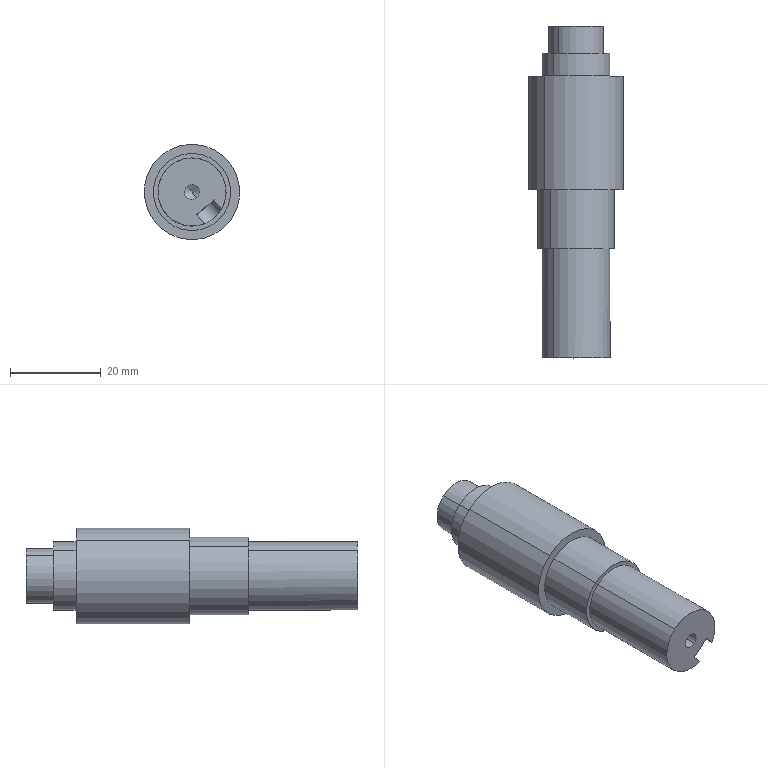Component | SolidWorks | CrankshaftOne-1_CrankshaftNo.1-1 | 1 solid | 28 faces | box 21 x 73 x 21 mm | volume 16750 mm3 | cylinder 15 | plane 9 | cone 4 | commonest cylinder face diameters 3.3 x4 15 x4 12 x2 21 x2 17 x2 5 x1 | material 5154-O, Bar (SS)
build123d program:
from build123d import *

# Parameters (mm, degrees)
CUT_EXTRUDE1_DEPTH    = 3
M4_TAPPED_HOLE1_D     = 3.3
M4_TAPPED_HOLE1_DEPTH = 20.5
M4_TAPPED_HOLE1_TIP   = 0.9914
M4_TAPPED_HOLE2_D     = 3.3
M4_TAPPED_HOLE2_DEPTH = 20.5
M4_TAPPED_HOLE2_TIP   = 0.9914


with BuildPart() as part:
    # Sketch1 → Revolve1 (revolve)
    with BuildSketch(Plane.XY, mode=Mode.PRIVATE) as revolve1_sk:
        Polygon((-85.215, 0), (-85.215, 7.5), (-61.215, 7.5), (-61.215, 8.5), (-48.215, 8.5), (-48.215, 10.5), (-23.215, 10.5), (-23.215, 7.5), (-18.215, 7.5), (-18.215, 6), (-12.215, 6), (-12.215, 0), align=None)
    revolve(revolve1_sk.sketch.rotate(Axis((-85.215, 0, 0), (1, 0, 0)), 90), axis=Axis((-85.215, 0, 0), (1, 0, 0)))

    # Sketch3 → Cut-Extrude1 (cut)
    with BuildSketch(Plane(origin=(-85.215, 0, -7.5), x_dir=(-1, 0, 0), z_dir=(0, 0, -1))):
        with BuildLine():
            Line((2.292, 2.5), (2.292, -2.5))
            Line((2.292, -2.5), (-19.5, -2.5))
            ThreePointArc((-19.5, -2.5), (-22, 0), (-19.5, 2.5))
            Line((-19.5, 2.5), (2.292, 2.5))
        make_face()
    extrude(amount=-CUT_EXTRUDE1_DEPTH, mode=Mode.SUBTRACT)

    # M4 Tapped Hole1
    with Locations(Plane.ZY.offset(85.215)):
        with Locations((0, 0)):
            Hole(M4_TAPPED_HOLE1_D / 2, depth=M4_TAPPED_HOLE1_DEPTH)
            with Locations((0, 0, -(M4_TAPPED_HOLE1_DEPTH + M4_TAPPED_HOLE1_TIP / 2))):  # 118° drill point
                Cone(0, M4_TAPPED_HOLE1_D / 2, M4_TAPPED_HOLE1_TIP, mode=Mode.SUBTRACT)

    # M4 Tapped Hole2
    with Locations(Plane(origin=(-12.215, 0, 0), x_dir=(0, 0, -1), z_dir=(1, 0, 0))):
        with Locations((0, 0)):
            Hole(M4_TAPPED_HOLE2_D / 2, depth=M4_TAPPED_HOLE2_DEPTH)
            with Locations((0, 0, -(M4_TAPPED_HOLE2_DEPTH + M4_TAPPED_HOLE2_TIP / 2))):  # 118° drill point
                Cone(0, M4_TAPPED_HOLE2_D / 2, M4_TAPPED_HOLE2_TIP, mode=Mode.SUBTRACT)


solid = part.part

# Placed as in the assembly
solid = solid.moved(Location((-199.914, 134.481, -166.507), (0, -41.206, 90)))
STEP:
#1=COLOUR_RGB('',0.7922,0.8196,0.9333);
#2=FILL_AREA_STYLE_COLOUR('',#1);
#3=FILL_AREA_STYLE('',(#2));
#4=SURFACE_STYLE_FILL_AREA(#3);
#5=SURFACE_SIDE_STYLE('',(#4));
#6=SURFACE_STYLE_USAGE(.BOTH.,#5);
#7=PRESENTATION_STYLE_ASSIGNMENT((#6));
#8=CARTESIAN_POINT('',(-7.913,4.007,-6.507));
#9=VERTEX_POINT('',#8);
#10=CARTESIAN_POINT('',(-7.828,4.007,-6.604));
#11=VERTEX_POINT('',#10);
#12=CARTESIAN_POINT('',(-7.871,4.007,-6.555));
#13=DIRECTION('',(-0.,1.,-0.));
#14=DIRECTION('',(0.6588,0.,-0.7523));
#15=AXIS2_PLACEMENT_3D('',#12,#13,#14);
#16=CIRCLE('',#15,0.06496);
#17=EDGE_CURVE('',#9,#11,#16,.T.);
#18=ORIENTED_EDGE('',*,*,#17,.F.);
#19=CARTESIAN_POINT('',(-7.913,4.814,-6.507));
#20=VERTEX_POINT('',#19);
#21=CARTESIAN_POINT('',(-7.913,4.814,-6.507));
#22=DIRECTION('',(-0.,1.,-0.));
#23=VECTOR('',#22,39.37);
#24=LINE('',#21,#23);
#25=EDGE_CURVE('',#9,#20,#24,.T.);
#26=ORIENTED_EDGE('',*,*,#25,.T.);
#27=CARTESIAN_POINT('',(-7.828,4.814,-6.604));
#28=VERTEX_POINT('',#27);
#29=CARTESIAN_POINT('',(-7.871,4.814,-6.555));
#30=DIRECTION('',(-0.,1.,-0.));
#31=DIRECTION('',(0.6588,0.,-0.7523));
#32=AXIS2_PLACEMENT_3D('',#29,#30,#31);
#33=CIRCLE('',#32,0.06496);
#34=EDGE_CURVE('',#20,#28,#33,.T.);
#35=ORIENTED_EDGE('',*,*,#34,.T.);
#36=CARTESIAN_POINT('',(-7.828,4.814,-6.604));
#37=DIRECTION('',(-0.,1.,-0.));
#38=VECTOR('',#37,39.37);
#39=LINE('',#36,#38);
#40=EDGE_CURVE('',#11,#28,#39,.T.);
#41=ORIENTED_EDGE('',*,*,#40,.F.);
#42=EDGE_LOOP('',(#18,#26,#35,#41));
#43=FACE_OUTER_BOUND('',#42,.T.);
#44=CARTESIAN_POINT('',(-7.871,4.814,-6.555));
#45=DIRECTION('',(-0.,1.,-0.));
#46=DIRECTION('',(0.6588,0.,-0.7523));
#47=AXIS2_PLACEMENT_3D('',#44,#45,#46);
#48=CYLINDRICAL_SURFACE('',#47,0.06496);
#49=ADVANCED_FACE('',(#43),#48,.F.);
#50=CARTESIAN_POINT('',(-7.871,3.968,-6.555));
#51=VERTEX_POINT('',#50);
#52=CARTESIAN_POINT('',(-7.828,4.007,-6.604));
#53=DIRECTION('',(0.5647,0.515,-0.6449));
#54=VECTOR('',#53,39.37);
#55=LINE('',#52,#54);
#56=EDGE_CURVE('',#51,#11,#55,.T.);
#57=ORIENTED_EDGE('',*,*,#56,.F.);
#58=CARTESIAN_POINT('',(-7.913,4.007,-6.507));
#59=DIRECTION('',(-0.5647,0.515,0.6449));
#60=VECTOR('',#59,39.37);
#61=LINE('',#58,#60);
#62=EDGE_CURVE('',#51,#9,#61,.T.);
#63=ORIENTED_EDGE('',*,*,#62,.T.);
#64=ORIENTED_EDGE('',*,*,#17,.T.);
#65=EDGE_LOOP('',(#57,#63,#64));
#66=FACE_OUTER_BOUND('',#65,.T.);
#67=CARTESIAN_POINT('',(-7.871,4.007,-6.555));
#68=DIRECTION('',(-0.,1.,-0.));
#69=DIRECTION('',(0.6588,0.,-0.7523));
#70=AXIS2_PLACEMENT_3D('',#67,#68,#69);
#71=CONICAL_SURFACE('',#70,0.06496,1.03);
#72=ADVANCED_FACE('',(#66),#71,.F.);
#73=CARTESIAN_POINT('',(-7.828,2.747,-6.604));
#74=VERTEX_POINT('',#73);
#75=CARTESIAN_POINT('',(-7.913,2.747,-6.507));
#76=VERTEX_POINT('',#75);
#77=CARTESIAN_POINT('',(-7.871,2.747,-6.555));
#78=DIRECTION('',(0.,-1.,0.));
#79=DIRECTION('',(-0.6588,0.,0.7523));
#80=AXIS2_PLACEMENT_3D('',#77,#78,#79);
#81=CIRCLE('',#80,0.06496);
#82=EDGE_CURVE('',#74,#76,#81,.T.);
#83=ORIENTED_EDGE('',*,*,#82,.F.);
#84=CARTESIAN_POINT('',(-7.828,1.94,-6.604));
#85=VERTEX_POINT('',#84);
#86=CARTESIAN_POINT('',(-7.828,1.94,-6.604));
#87=DIRECTION('',(0.,-1.,0.));
#88=VECTOR('',#87,39.37);
#89=LINE('',#86,#88);
#90=EDGE_CURVE('',#74,#85,#89,.T.);
#91=ORIENTED_EDGE('',*,*,#90,.T.);
#92=CARTESIAN_POINT('',(-7.913,1.94,-6.507));
#93=VERTEX_POINT('',#92);
#94=CARTESIAN_POINT('',(-7.871,1.94,-6.555));
#95=DIRECTION('',(0.,-1.,0.));
#96=DIRECTION('',(-0.6588,0.,0.7523));
#97=AXIS2_PLACEMENT_3D('',#94,#95,#96);
#98=CIRCLE('',#97,0.06496);
#99=EDGE_CURVE('',#85,#93,#98,.T.);
#100=ORIENTED_EDGE('',*,*,#99,.T.);
#101=CARTESIAN_POINT('',(-7.913,1.94,-6.507));
#102=DIRECTION('',(0.,-1.,0.));
#103=VECTOR('',#102,39.37);
#104=LINE('',#101,#103);
#105=EDGE_CURVE('',#76,#93,#104,.T.);
#106=ORIENTED_EDGE('',*,*,#105,.F.);
#107=EDGE_LOOP('',(#83,#91,#100,#106));
#108=FACE_OUTER_BOUND('',#107,.T.);
#109=CARTESIAN_POINT('',(-7.871,1.94,-6.555));
#110=DIRECTION('',(0.,-1.,0.));
#111=DIRECTION('',(-0.6588,0.,0.7523));
#112=AXIS2_PLACEMENT_3D('',#109,#110,#111);
#113=CYLINDRICAL_SURFACE('',#112,0.06496);
#114=ADVANCED_FACE('',(#108),#113,.F.);
#115=CARTESIAN_POINT('',(-7.871,2.786,-6.555));
#116=VERTEX_POINT('',#115);
#117=CARTESIAN_POINT('',(-7.913,2.747,-6.507));
#118=DIRECTION('',(-0.5647,-0.515,0.6449));
#119=VECTOR('',#118,39.37);
#120=LINE('',#117,#119);
#121=EDGE_CURVE('',#116,#76,#120,.T.);
#122=ORIENTED_EDGE('',*,*,#121,.F.);
#123=CARTESIAN_POINT('',(-7.828,2.747,-6.604));
#124=DIRECTION('',(0.5647,-0.515,-0.6449));
#125=VECTOR('',#124,39.37);
#126=LINE('',#123,#125);
#127=EDGE_CURVE('',#116,#74,#126,.T.);
#128=ORIENTED_EDGE('',*,*,#127,.T.);
#129=ORIENTED_EDGE('',*,*,#82,.T.);
#130=EDGE_LOOP('',(#122,#128,#129));
#131=FACE_OUTER_BOUND('',#130,.T.);
#132=CARTESIAN_POINT('',(-7.871,2.747,-6.555));
#133=DIRECTION('',(0.,-1.,0.));
#134=DIRECTION('',(-0.6588,0.,0.7523));
#135=AXIS2_PLACEMENT_3D('',#132,#133,#134);
#136=CONICAL_SURFACE('',#135,0.06496,1.03);
#137=ADVANCED_FACE('',(#131),#136,.F.);
#138=CARTESIAN_POINT('',(-8.026,4.814,-6.378));
#139=VERTEX_POINT('',#138);
#140=CARTESIAN_POINT('',(-7.715,4.814,-6.733));
#141=VERTEX_POINT('',#140);
#142=CARTESIAN_POINT('',(-7.871,4.814,-6.555));
#143=DIRECTION('',(0.,-1.,0.));
#144=DIRECTION('',(-0.6588,0.,0.7523));
#145=AXIS2_PLACEMENT_3D('',#142,#143,#144);
#146=CIRCLE('',#145,0.2362);
#147=EDGE_CURVE('',#139,#141,#146,.T.);
#148=ORIENTED_EDGE('',*,*,#147,.T.);
#149=CARTESIAN_POINT('',(-7.715,4.577,-6.733));
#150=VERTEX_POINT('',#149);
#151=CARTESIAN_POINT('',(-7.715,1.94,-6.733));
#152=DIRECTION('',(0.,-1.,0.));
#153=VECTOR('',#152,39.37);
#154=LINE('',#151,#153);
#155=EDGE_CURVE('',#141,#150,#154,.T.);
#156=ORIENTED_EDGE('',*,*,#155,.T.);
#157=CARTESIAN_POINT('',(-8.026,4.577,-6.378));
#158=VERTEX_POINT('',#157);
#159=CARTESIAN_POINT('',(-7.871,4.577,-6.555));
#160=DIRECTION('',(0.,-1.,0.));
#161=DIRECTION('',(-0.6588,0.,0.7523));
#162=AXIS2_PLACEMENT_3D('',#159,#160,#161);
#163=CIRCLE('',#162,0.2362);
#164=EDGE_CURVE('',#158,#150,#163,.T.);
#165=ORIENTED_EDGE('',*,*,#164,.F.);
#166=CARTESIAN_POINT('',(-8.026,1.94,-6.378));
#167=DIRECTION('',(0.,-1.,0.));
#168=VECTOR('',#167,39.37);
#169=LINE('',#166,#168);
#170=EDGE_CURVE('',#139,#158,#169,.T.);
#171=ORIENTED_EDGE('',*,*,#170,.F.);
#172=EDGE_LOOP('',(#148,#156,#165,#171));
#173=FACE_OUTER_BOUND('',#172,.T.);
#174=CARTESIAN_POINT('',(-7.871,1.94,-6.555));
#175=DIRECTION('',(0.,-1.,0.));
#176=DIRECTION('',(-0.6588,0.,0.7523));
#177=AXIS2_PLACEMENT_3D('',#174,#175,#176);
#178=CYLINDRICAL_SURFACE('',#177,0.2362);
#179=ADVANCED_FACE('',(#173),#178,.T.);
#180=CARTESIAN_POINT('',(-8.065,4.577,-6.333));
#181=VERTEX_POINT('',#180);
#182=CARTESIAN_POINT('',(-7.676,4.577,-6.778));
#183=VERTEX_POINT('',#182);
#184=CARTESIAN_POINT('',(-7.871,4.577,-6.555));
#185=DIRECTION('',(0.,-1.,0.));
#186=DIRECTION('',(-0.6588,0.,0.7523));
#187=AXIS2_PLACEMENT_3D('',#184,#185,#186);
#188=CIRCLE('',#187,0.2953);
#189=EDGE_CURVE('',#181,#183,#188,.T.);
#190=ORIENTED_EDGE('',*,*,#189,.T.);
#191=CARTESIAN_POINT('',(-7.676,4.381,-6.778));
#192=VERTEX_POINT('',#191);
#193=CARTESIAN_POINT('',(-7.676,1.94,-6.778));
#194=DIRECTION('',(0.,-1.,0.));
#195=VECTOR('',#194,39.37);
#196=LINE('',#193,#195);
#197=EDGE_CURVE('',#183,#192,#196,.T.);
#198=ORIENTED_EDGE('',*,*,#197,.T.);
#199=CARTESIAN_POINT('',(-8.065,4.381,-6.333));
#200=VERTEX_POINT('',#199);
#201=CARTESIAN_POINT('',(-7.871,4.381,-6.555));
#202=DIRECTION('',(0.,-1.,0.));
#203=DIRECTION('',(-0.6588,0.,0.7523));
#204=AXIS2_PLACEMENT_3D('',#201,#202,#203);
#205=CIRCLE('',#204,0.2953);
#206=EDGE_CURVE('',#200,#192,#205,.T.);
#207=ORIENTED_EDGE('',*,*,#206,.F.);
#208=CARTESIAN_POINT('',(-8.065,1.94,-6.333));
#209=DIRECTION('',(0.,-1.,0.));
#210=VECTOR('',#209,39.37);
#211=LINE('',#208,#210);
#212=EDGE_CURVE('',#181,#200,#211,.T.);
#213=ORIENTED_EDGE('',*,*,#212,.F.);
#214=EDGE_LOOP('',(#190,#198,#207,#213));
#215=FACE_OUTER_BOUND('',#214,.T.);
#216=CARTESIAN_POINT('',(-7.871,1.94,-6.555));
#217=DIRECTION('',(0.,-1.,0.));
#218=DIRECTION('',(-0.6588,0.,0.7523));
#219=AXIS2_PLACEMENT_3D('',#216,#217,#218);
#220=CYLINDRICAL_SURFACE('',#219,0.2953);
#221=ADVANCED_FACE('',(#215),#220,.T.);
#222=CARTESIAN_POINT('',(-8.143,4.381,-6.244));
#223=VERTEX_POINT('',#222);
#224=CARTESIAN_POINT('',(-7.598,4.381,-6.866));
#225=VERTEX_POINT('',#224);
#226=CARTESIAN_POINT('',(-7.871,4.381,-6.555));
#227=DIRECTION('',(0.,-1.,0.));
#228=DIRECTION('',(-0.6588,0.,0.7523));
#229=AXIS2_PLACEMENT_3D('',#226,#227,#228);
#230=CIRCLE('',#229,0.4134);
#231=EDGE_CURVE('',#223,#225,#230,.T.);
#232=ORIENTED_EDGE('',*,*,#231,.T.);
#233=CARTESIAN_POINT('',(-7.598,3.396,-6.866));
#234=VERTEX_POINT('',#233);
#235=CARTESIAN_POINT('',(-7.598,1.94,-6.866));
#236=DIRECTION('',(0.,-1.,0.));
#237=VECTOR('',#236,39.37);
#238=LINE('',#235,#237);
#239=EDGE_CURVE('',#225,#234,#238,.T.);
#240=ORIENTED_EDGE('',*,*,#239,.T.);
#241=CARTESIAN_POINT('',(-8.143,3.396,-6.244));
#242=VERTEX_POINT('',#241);
#243=CARTESIAN_POINT('',(-7.871,3.396,-6.555));
#244=DIRECTION('',(0.,-1.,0.));
#245=DIRECTION('',(-0.6588,0.,0.7523));
#246=AXIS2_PLACEMENT_3D('',#243,#244,#245);
#247=CIRCLE('',#246,0.4134);
#248=EDGE_CURVE('',#242,#234,#247,.T.);
#249=ORIENTED_EDGE('',*,*,#248,.F.);
#250=CARTESIAN_POINT('',(-8.143,1.94,-6.244));
#251=DIRECTION('',(0.,-1.,0.));
#252=VECTOR('',#251,39.37);
#253=LINE('',#250,#252);
#254=EDGE_CURVE('',#223,#242,#253,.T.);
#255=ORIENTED_EDGE('',*,*,#254,.F.);
#256=EDGE_LOOP('',(#232,#240,#249,#255));
#257=FACE_OUTER_BOUND('',#256,.T.);
#258=CARTESIAN_POINT('',(-7.871,1.94,-6.555));
#259=DIRECTION('',(0.,-1.,0.));
#260=DIRECTION('',(-0.6588,0.,0.7523));
#261=AXIS2_PLACEMENT_3D('',#258,#259,#260);
#262=CYLINDRICAL_SURFACE('',#261,0.4134);
#263=ADVANCED_FACE('',(#257),#262,.T.);
#264=CARTESIAN_POINT('',(-8.091,3.396,-6.304));
#265=VERTEX_POINT('',#264);
#266=CARTESIAN_POINT('',(-7.65,3.396,-6.807));
#267=VERTEX_POINT('',#266);
#268=CARTESIAN_POINT('',(-7.871,3.396,-6.555));
#269=DIRECTION('',(0.,-1.,0.));
#270=DIRECTION('',(-0.6588,0.,0.7523));
#271=AXIS2_PLACEMENT_3D('',#268,#269,#270);
#272=CIRCLE('',#271,0.3346);
#273=EDGE_CURVE('',#265,#267,#272,.T.);
#274=ORIENTED_EDGE('',*,*,#273,.T.);
#275=CARTESIAN_POINT('',(-7.65,2.884,-6.807));
#276=VERTEX_POINT('',#275);
#277=CARTESIAN_POINT('',(-7.65,1.94,-6.807));
#278=DIRECTION('',(0.,-1.,0.));
#279=VECTOR('',#278,39.37);
#280=LINE('',#277,#279);
#281=EDGE_CURVE('',#267,#276,#280,.T.);
#282=ORIENTED_EDGE('',*,*,#281,.T.);
#283=CARTESIAN_POINT('',(-8.091,2.884,-6.304));
#284=VERTEX_POINT('',#283);
#285=CARTESIAN_POINT('',(-7.871,2.884,-6.555));
#286=DIRECTION('',(0.,-1.,0.));
#287=DIRECTION('',(-0.6588,0.,0.7523));
#288=AXIS2_PLACEMENT_3D('',#285,#286,#287);
#289=CIRCLE('',#288,0.3346);
#290=EDGE_CURVE('',#284,#276,#289,.T.);
#291=ORIENTED_EDGE('',*,*,#290,.F.);
#292=CARTESIAN_POINT('',(-8.091,1.94,-6.304));
#293=DIRECTION('',(0.,-1.,0.));
#294=VECTOR('',#293,39.37);
#295=LINE('',#292,#294);
#296=EDGE_CURVE('',#265,#284,#295,.T.);
#297=ORIENTED_EDGE('',*,*,#296,.F.);
#298=EDGE_LOOP('',(#274,#282,#291,#297));
#299=FACE_OUTER_BOUND('',#298,.T.);
#300=CARTESIAN_POINT('',(-7.871,1.94,-6.555));
#301=DIRECTION('',(0.,-1.,0.));
#302=DIRECTION('',(-0.6588,0.,0.7523));
#303=AXIS2_PLACEMENT_3D('',#300,#301,#302);
#304=CYLINDRICAL_SURFACE('',#303,0.3346);
#305=ADVANCED_FACE('',(#299),#304,.T.);
#306=CARTESIAN_POINT('',(-8.065,2.884,-6.333));
#307=VERTEX_POINT('',#306);
#308=CARTESIAN_POINT('',(-7.676,2.884,-6.778));
#309=VERTEX_POINT('',#308);
#310=CARTESIAN_POINT('',(-7.871,2.884,-6.555));
#311=DIRECTION('',(0.,-1.,0.));
#312=DIRECTION('',(-0.6588,0.,0.7523));
#313=AXIS2_PLACEMENT_3D('',#310,#311,#312);
#314=CIRCLE('',#313,0.2953);
#315=EDGE_CURVE('',#307,#309,#314,.T.);
#316=ORIENTED_EDGE('',*,*,#315,.T.);
#317=CARTESIAN_POINT('',(-7.676,2.806,-6.778));
#318=VERTEX_POINT('',#317);
#319=CARTESIAN_POINT('',(-7.676,1.94,-6.778));
#320=DIRECTION('',(0.,-1.,0.));
#321=VECTOR('',#320,39.37);
#322=LINE('',#319,#321);
#323=EDGE_CURVE('',#309,#318,#322,.T.);
#324=ORIENTED_EDGE('',*,*,#323,.T.);
#325=CARTESIAN_POINT('',(-7.761,2.707,-6.83));
#326=VERTEX_POINT('',#325);
#327=CARTESIAN_POINT('',(-7.676,2.806,-6.778));
#328=CARTESIAN_POINT('',(-7.681,2.806,-6.782));
#329=CARTESIAN_POINT('',(-7.686,2.805,-6.786));
#330=CARTESIAN_POINT('',(-7.696,2.803,-6.794));
#331=CARTESIAN_POINT('',(-7.701,2.801,-6.797));
#332=CARTESIAN_POINT('',(-7.711,2.796,-6.804));
#333=CARTESIAN_POINT('',(-7.716,2.793,-6.807));
#334=CARTESIAN_POINT('',(-7.725,2.786,-6.813));
#335=CARTESIAN_POINT('',(-7.73,2.781,-6.815));
#336=CARTESIAN_POINT('',(-7.738,2.772,-6.819));
#337=CARTESIAN_POINT('',(-7.742,2.767,-6.821));
#338=CARTESIAN_POINT('',(-7.749,2.757,-6.824));
#339=CARTESIAN_POINT('',(-7.752,2.751,-6.826));
#340=CARTESIAN_POINT('',(-7.756,2.739,-6.828));
#341=CARTESIAN_POINT('',(-7.758,2.733,-6.828));
#342=CARTESIAN_POINT('',(-7.761,2.72,-6.829));
#343=CARTESIAN_POINT('',(-7.761,2.714,-6.83));
#344=CARTESIAN_POINT('',(-7.761,2.707,-6.83));
#345=B_SPLINE_CURVE_WITH_KNOTS('',3,(#327,#328,#329,#330,#331,#332,#333,#334,#335,#336,#337,#338,#339,#340,#341,#342,#343,#344),.UNSPECIFIED.,.F.,.F.,(4,2,2,2,2,2,2,2,4),(0.003937,0.004429,0.004921,0.005412,0.005904,0.006395,0.006887,0.007378,0.00787),.UNSPECIFIED.);
#346=EDGE_CURVE('',#318,#326,#345,.T.);
#347=ORIENTED_EDGE('',*,*,#346,.T.);
#348=CARTESIAN_POINT('',(-7.761,1.94,-6.83));
#349=VERTEX_POINT('',#348);
#350=CARTESIAN_POINT('',(-7.761,1.94,-6.83));
#351=DIRECTION('',(0.,-1.,0.));
#352=VECTOR('',#351,39.37);
#353=LINE('',#350,#352);
#354=EDGE_CURVE('',#326,#349,#353,.T.);
#355=ORIENTED_EDGE('',*,*,#354,.T.);
#356=CARTESIAN_POINT('',(-8.065,1.94,-6.333));
#357=VERTEX_POINT('',#356);
#358=CARTESIAN_POINT('',(-7.871,1.94,-6.555));
#359=DIRECTION('',(0.,-1.,0.));
#360=DIRECTION('',(-0.6588,0.,0.7523));
#361=AXIS2_PLACEMENT_3D('',#358,#359,#360);
#362=CIRCLE('',#361,0.2953);
#363=EDGE_CURVE('',#357,#349,#362,.T.);
#364=ORIENTED_EDGE('',*,*,#363,.F.);
#365=CARTESIAN_POINT('',(-8.065,1.94,-6.333));
#366=DIRECTION('',(0.,-1.,0.));
#367=VECTOR('',#366,39.37);
#368=LINE('',#365,#367);
#369=EDGE_CURVE('',#307,#357,#368,.T.);
#370=ORIENTED_EDGE('',*,*,#369,.F.);
#371=EDGE_LOOP('',(#316,#324,#347,#355,#364,#370));
#372=FACE_OUTER_BOUND('',#371,.T.);
#373=CARTESIAN_POINT('',(-7.871,1.94,-6.555));
#374=DIRECTION('',(0.,-1.,0.));
#375=DIRECTION('',(-0.6588,0.,0.7523));
#376=AXIS2_PLACEMENT_3D('',#373,#374,#375);
#377=CYLINDRICAL_SURFACE('',#376,0.2953);
#378=ADVANCED_FACE('',(#372),#377,.T.);
#379=CARTESIAN_POINT('',(-7.871,1.94,-6.555));
#380=DIRECTION('',(0.,-1.,0.));
#381=DIRECTION('',(-0.6588,0.,0.7523));
#382=AXIS2_PLACEMENT_3D('',#379,#380,#381);
#383=CIRCLE('',#382,0.06496);
#384=EDGE_CURVE('',#93,#85,#383,.T.);
#385=ORIENTED_EDGE('',*,*,#384,.F.);
#386=ORIENTED_EDGE('',*,*,#99,.F.);
#387=EDGE_LOOP('',(#385,#386));
#388=FACE_BOUND('',#387,.T.);
#389=CARTESIAN_POINT('',(-7.613,1.94,-6.7));
#390=VERTEX_POINT('',#389);
#391=CARTESIAN_POINT('',(-7.871,1.94,-6.555));
#392=DIRECTION('',(0.,-1.,0.));
#393=DIRECTION('',(-0.6588,0.,0.7523));
#394=AXIS2_PLACEMENT_3D('',#391,#392,#393);
#395=CIRCLE('',#394,0.2953);
#396=EDGE_CURVE('',#390,#357,#395,.T.);
#397=ORIENTED_EDGE('',*,*,#396,.T.);
#398=ORIENTED_EDGE('',*,*,#363,.T.);
#399=CARTESIAN_POINT('',(-7.828,1.94,-6.754));
#400=VERTEX_POINT('',#399);
#401=CARTESIAN_POINT('',(-7.945,1.94,-6.62));
#402=DIRECTION('',(-0.6588,-0.,0.7523));
#403=VECTOR('',#402,39.37);
#404=LINE('',#401,#403);
#405=EDGE_CURVE('',#349,#400,#404,.T.);
#406=ORIENTED_EDGE('',*,*,#405,.T.);
#407=CARTESIAN_POINT('',(-7.68,1.94,-6.624));
#408=VERTEX_POINT('',#407);
#409=CARTESIAN_POINT('',(-7.754,1.94,-6.689));
#410=DIRECTION('',(-0.7523,-0.,-0.6588));
#411=VECTOR('',#410,39.37);
#412=LINE('',#409,#411);
#413=EDGE_CURVE('',#408,#400,#412,.T.);
#414=ORIENTED_EDGE('',*,*,#413,.F.);
#415=CARTESIAN_POINT('',(-7.797,1.94,-6.491));
#416=DIRECTION('',(0.6588,0.,-0.7523));
#417=VECTOR('',#416,39.37);
#418=LINE('',#415,#417);
#419=EDGE_CURVE('',#408,#390,#418,.T.);
#420=ORIENTED_EDGE('',*,*,#419,.T.);
#421=EDGE_LOOP('',(#397,#398,#406,#414,#420));
#422=FACE_OUTER_BOUND('',#421,.T.);
#423=CARTESIAN_POINT('',(-7.871,1.94,-6.555));
#424=DIRECTION('',(-0.,1.,-0.));
#425=DIRECTION('',(0.6588,0.,-0.7523));
#426=AXIS2_PLACEMENT_3D('',#423,#424,#425);
#427=PLANE('',#426);
#428=ADVANCED_FACE('',(#388,#422),#427,.F.);
#429=ORIENTED_EDGE('',*,*,#323,.F.);
#430=CARTESIAN_POINT('',(-7.871,2.884,-6.555));
#431=DIRECTION('',(0.,-1.,0.));
#432=DIRECTION('',(-0.6588,0.,0.7523));
#433=AXIS2_PLACEMENT_3D('',#430,#431,#432);
#434=CIRCLE('',#433,0.2953);
#435=EDGE_CURVE('',#309,#307,#434,.T.);
#436=ORIENTED_EDGE('',*,*,#435,.T.);
#437=ORIENTED_EDGE('',*,*,#369,.T.);
#438=ORIENTED_EDGE('',*,*,#396,.F.);
#439=CARTESIAN_POINT('',(-7.613,2.707,-6.7));
#440=VERTEX_POINT('',#439);
#441=CARTESIAN_POINT('',(-7.613,1.94,-6.7));
#442=DIRECTION('',(-0.,1.,-0.));
#443=VECTOR('',#442,39.37);
#444=LINE('',#441,#443);
#445=EDGE_CURVE('',#390,#440,#444,.T.);
#446=ORIENTED_EDGE('',*,*,#445,.T.);
#447=CARTESIAN_POINT('',(-7.613,2.707,-6.7));
#448=CARTESIAN_POINT('',(-7.613,2.714,-6.7));
#449=CARTESIAN_POINT('',(-7.614,2.72,-6.701));
#450=CARTESIAN_POINT('',(-7.615,2.733,-6.703));
#451=CARTESIAN_POINT('',(-7.616,2.739,-6.705));
#452=CARTESIAN_POINT('',(-7.619,2.751,-6.709));
#453=CARTESIAN_POINT('',(-7.62,2.757,-6.712));
#454=CARTESIAN_POINT('',(-7.624,2.767,-6.718));
#455=CARTESIAN_POINT('',(-7.627,2.772,-6.722));
#456=CARTESIAN_POINT('',(-7.635,2.786,-6.733));
#457=CARTESIAN_POINT('',(-7.641,2.793,-6.742));
#458=CARTESIAN_POINT('',(-7.653,2.801,-6.755));
#459=CARTESIAN_POINT('',(-7.658,2.803,-6.76));
#460=CARTESIAN_POINT('',(-7.667,2.805,-6.769));
#461=CARTESIAN_POINT('',(-7.671,2.806,-6.773));
#462=CARTESIAN_POINT('',(-7.676,2.806,-6.778));
#463=B_SPLINE_CURVE_WITH_KNOTS('',3,(#447,#448,#449,#450,#451,#452,#453,#454,#455,#456,#457,#458,#459,#460,#461,#462),.UNSPECIFIED.,.F.,.F.,(4,2,2,2,2,2,2,4),(0.,0.0004922,0.0009844,0.001477,0.001969,0.002953,0.003445,0.003937),.UNSPECIFIED.);
#464=EDGE_CURVE('',#440,#318,#463,.T.);
#465=ORIENTED_EDGE('',*,*,#464,.T.);
#466=EDGE_LOOP('',(#429,#436,#437,#438,#446,#465));
#467=FACE_OUTER_BOUND('',#466,.T.);
#468=CARTESIAN_POINT('',(-7.871,1.94,-6.555));
#469=DIRECTION('',(0.,-1.,0.));
#470=DIRECTION('',(-0.6588,0.,0.7523));
#471=AXIS2_PLACEMENT_3D('',#468,#469,#470);
#472=CYLINDRICAL_SURFACE('',#471,0.2953);
#473=ADVANCED_FACE('',(#467),#472,.T.);
#474=ORIENTED_EDGE('',*,*,#315,.F.);
#475=ORIENTED_EDGE('',*,*,#435,.F.);
#476=EDGE_LOOP('',(#474,#475));
#477=FACE_BOUND('',#476,.T.);
#478=ORIENTED_EDGE('',*,*,#290,.T.);
#479=CARTESIAN_POINT('',(-7.871,2.884,-6.555));
#480=DIRECTION('',(0.,-1.,0.));
#481=DIRECTION('',(-0.6588,0.,0.7523));
#482=AXIS2_PLACEMENT_3D('',#479,#480,#481);
#483=CIRCLE('',#482,0.3346);
#484=EDGE_CURVE('',#276,#284,#483,.T.);
#485=ORIENTED_EDGE('',*,*,#484,.T.);
#486=EDGE_LOOP('',(#478,#485));
#487=FACE_OUTER_BOUND('',#486,.T.);
#488=CARTESIAN_POINT('',(-8.093,2.884,-6.75));
#489=DIRECTION('',(-0.,1.,-0.));
#490=DIRECTION('',(0.6588,0.,-0.7523));
#491=AXIS2_PLACEMENT_3D('',#488,#489,#490);
#492=PLANE('',#491);
#493=ADVANCED_FACE('',(#477,#487),#492,.F.);
#494=ORIENTED_EDGE('',*,*,#281,.F.);
#495=CARTESIAN_POINT('',(-7.871,3.396,-6.555));
#496=DIRECTION('',(0.,-1.,0.));
#497=DIRECTION('',(-0.6588,0.,0.7523));
#498=AXIS2_PLACEMENT_3D('',#495,#496,#497);
#499=CIRCLE('',#498,0.3346);
#500=EDGE_CURVE('',#267,#265,#499,.T.);
#501=ORIENTED_EDGE('',*,*,#500,.T.);
#502=ORIENTED_EDGE('',*,*,#296,.T.);
#503=ORIENTED_EDGE('',*,*,#484,.F.);
#504=EDGE_LOOP('',(#494,#501,#502,#503));
#505=FACE_OUTER_BOUND('',#504,.T.);
#506=CARTESIAN_POINT('',(-7.871,1.94,-6.555));
#507=DIRECTION('',(0.,-1.,0.));
#508=DIRECTION('',(-0.6588,0.,0.7523));
#509=AXIS2_PLACEMENT_3D('',#506,#507,#508);
#510=CYLINDRICAL_SURFACE('',#509,0.3346);
#511=ADVANCED_FACE('',(#505),#510,.T.);
#512=ORIENTED_EDGE('',*,*,#273,.F.);
#513=ORIENTED_EDGE('',*,*,#500,.F.);
#514=EDGE_LOOP('',(#512,#513));
#515=FACE_BOUND('',#514,.T.);
#516=ORIENTED_EDGE('',*,*,#248,.T.);
#517=CARTESIAN_POINT('',(-7.871,3.396,-6.555));
#518=DIRECTION('',(0.,-1.,0.));
#519=DIRECTION('',(-0.6588,0.,0.7523));
#520=AXIS2_PLACEMENT_3D('',#517,#518,#519);
#521=CIRCLE('',#520,0.4134);
#522=EDGE_CURVE('',#234,#242,#521,.T.);
#523=ORIENTED_EDGE('',*,*,#522,.T.);
#524=EDGE_LOOP('',(#516,#523));
#525=FACE_OUTER_BOUND('',#524,.T.);
#526=CARTESIAN_POINT('',(-8.122,3.396,-6.776));
#527=DIRECTION('',(-0.,1.,-0.));
#528=DIRECTION('',(0.6588,0.,-0.7523));
#529=AXIS2_PLACEMENT_3D('',#526,#527,#528);
#530=PLANE('',#529);
#531=ADVANCED_FACE('',(#515,#525),#530,.F.);
#532=ORIENTED_EDGE('',*,*,#239,.F.);
#533=CARTESIAN_POINT('',(-7.871,4.381,-6.555));
#534=DIRECTION('',(0.,-1.,0.));
#535=DIRECTION('',(-0.6588,0.,0.7523));
#536=AXIS2_PLACEMENT_3D('',#533,#534,#535);
#537=CIRCLE('',#536,0.4134);
#538=EDGE_CURVE('',#225,#223,#537,.T.);
#539=ORIENTED_EDGE('',*,*,#538,.T.);
#540=ORIENTED_EDGE('',*,*,#254,.T.);
#541=ORIENTED_EDGE('',*,*,#522,.F.);
#542=EDGE_LOOP('',(#532,#539,#540,#541));
#543=FACE_OUTER_BOUND('',#542,.T.);
#544=CARTESIAN_POINT('',(-7.871,1.94,-6.555));
#545=DIRECTION('',(0.,-1.,0.));
#546=DIRECTION('',(-0.6588,0.,0.7523));
#547=AXIS2_PLACEMENT_3D('',#544,#545,#546);
#548=CYLINDRICAL_SURFACE('',#547,0.4134);
#549=ADVANCED_FACE('',(#543),#548,.T.);
#550=ORIENTED_EDGE('',*,*,#231,.F.);
#551=ORIENTED_EDGE('',*,*,#538,.F.);
#552=EDGE_LOOP('',(#550,#551));
#553=FACE_OUTER_BOUND('',#552,.T.);
#554=ORIENTED_EDGE('',*,*,#206,.T.);
#555=CARTESIAN_POINT('',(-7.871,4.381,-6.555));
#556=DIRECTION('',(0.,-1.,0.));
#557=DIRECTION('',(-0.6588,0.,0.7523));
#558=AXIS2_PLACEMENT_3D('',#555,#556,#557);
#559=CIRCLE('',#558,0.2953);
#560=EDGE_CURVE('',#192,#200,#559,.T.);
#561=ORIENTED_EDGE('',*,*,#560,.T.);
#562=EDGE_LOOP('',(#554,#561));
#563=FACE_BOUND('',#562,.T.);
#564=CARTESIAN_POINT('',(-8.182,4.381,-6.828));
#565=DIRECTION('',(0.,-1.,0.));
#566=DIRECTION('',(-0.6588,-0.,0.7523));
#567=AXIS2_PLACEMENT_3D('',#564,#565,#566);
#568=PLANE('',#567);
#569=ADVANCED_FACE('',(#553,#563),#568,.F.);
#570=ORIENTED_EDGE('',*,*,#197,.F.);
#571=CARTESIAN_POINT('',(-7.871,4.577,-6.555));
#572=DIRECTION('',(0.,-1.,0.));
#573=DIRECTION('',(-0.6588,0.,0.7523));
#574=AXIS2_PLACEMENT_3D('',#571,#572,#573);
#575=CIRCLE('',#574,0.2953);
#576=EDGE_CURVE('',#183,#181,#575,.T.);
#577=ORIENTED_EDGE('',*,*,#576,.T.);
#578=ORIENTED_EDGE('',*,*,#212,.T.);
#579=ORIENTED_EDGE('',*,*,#560,.F.);
#580=EDGE_LOOP('',(#570,#577,#578,#579));
#581=FACE_OUTER_BOUND('',#580,.T.);
#582=CARTESIAN_POINT('',(-7.871,1.94,-6.555));
#583=DIRECTION('',(0.,-1.,0.));
#584=DIRECTION('',(-0.6588,0.,0.7523));
#585=AXIS2_PLACEMENT_3D('',#582,#583,#584);
#586=CYLINDRICAL_SURFACE('',#585,0.2953);
#587=ADVANCED_FACE('',(#581),#586,.T.);
#588=ORIENTED_EDGE('',*,*,#189,.F.);
#589=ORIENTED_EDGE('',*,*,#576,.F.);
#590=EDGE_LOOP('',(#588,#589));
#591=FACE_OUTER_BOUND('',#590,.T.);
#592=ORIENTED_EDGE('',*,*,#164,.T.);
#593=CARTESIAN_POINT('',(-7.871,4.577,-6.555));
#594=DIRECTION('',(0.,-1.,0.));
#595=DIRECTION('',(-0.6588,0.,0.7523));
#596=AXIS2_PLACEMENT_3D('',#593,#594,#595);
#597=CIRCLE('',#596,0.2362);
#598=EDGE_CURVE('',#150,#158,#597,.T.);
#599=ORIENTED_EDGE('',*,*,#598,.T.);
#600=EDGE_LOOP('',(#592,#599));
#601=FACE_BOUND('',#600,.T.);
#602=CARTESIAN_POINT('',(-8.093,4.577,-6.75));
#603=DIRECTION('',(0.,-1.,0.));
#604=DIRECTION('',(-0.6588,-0.,0.7523));
#605=AXIS2_PLACEMENT_3D('',#602,#603,#604);
#606=PLANE('',#605);
#607=ADVANCED_FACE('',(#591,#601),#606,.F.);
#608=ORIENTED_EDGE('',*,*,#155,.F.);
#609=CARTESIAN_POINT('',(-7.871,4.814,-6.555));
#610=DIRECTION('',(0.,-1.,0.));
#611=DIRECTION('',(-0.6588,0.,0.7523));
#612=AXIS2_PLACEMENT_3D('',#609,#610,#611);
#613=CIRCLE('',#612,0.2362);
#614=EDGE_CURVE('',#141,#139,#613,.T.);
#615=ORIENTED_EDGE('',*,*,#614,.T.);
#616=ORIENTED_EDGE('',*,*,#170,.T.);
#617=ORIENTED_EDGE('',*,*,#598,.F.);
#618=EDGE_LOOP('',(#608,#615,#616,#617));
#619=FACE_OUTER_BOUND('',#618,.T.);
#620=CARTESIAN_POINT('',(-7.871,1.94,-6.555));
#621=DIRECTION('',(0.,-1.,0.));
#622=DIRECTION('',(-0.6588,0.,0.7523));
#623=AXIS2_PLACEMENT_3D('',#620,#621,#622);
#624=CYLINDRICAL_SURFACE('',#623,0.2362);
#625=ADVANCED_FACE('',(#619),#624,.T.);
#626=CARTESIAN_POINT('',(-7.871,4.814,-6.555));
#627=DIRECTION('',(-0.,1.,-0.));
#628=DIRECTION('',(0.6588,0.,-0.7523));
#629=AXIS2_PLACEMENT_3D('',#626,#627,#628);
#630=CIRCLE('',#629,0.06496);
#631=EDGE_CURVE('',#28,#20,#630,.T.);
#632=ORIENTED_EDGE('',*,*,#631,.F.);
#633=ORIENTED_EDGE('',*,*,#34,.F.);
#634=EDGE_LOOP('',(#632,#633));
#635=FACE_BOUND('',#634,.T.);
#636=ORIENTED_EDGE('',*,*,#147,.F.);
#637=ORIENTED_EDGE('',*,*,#614,.F.);
#638=EDGE_LOOP('',(#636,#637));
#639=FACE_OUTER_BOUND('',#638,.T.);
#640=CARTESIAN_POINT('',(-8.048,4.814,-6.711));
#641=DIRECTION('',(0.,-1.,0.));
#642=DIRECTION('',(-0.6588,-0.,0.7523));
#643=AXIS2_PLACEMENT_3D('',#640,#641,#642);
#644=PLANE('',#643);
#645=ADVANCED_FACE('',(#635,#639),#644,.F.);
#646=ORIENTED_EDGE('',*,*,#413,.T.);
#647=CARTESIAN_POINT('',(-7.828,2.707,-6.754));
#648=VERTEX_POINT('',#647);
#649=CARTESIAN_POINT('',(-7.828,2.707,-6.754));
#650=DIRECTION('',(-0.,1.,-0.));
#651=VECTOR('',#650,39.37);
#652=LINE('',#649,#651);
#653=EDGE_CURVE('',#400,#648,#652,.T.);
#654=ORIENTED_EDGE('',*,*,#653,.T.);
#655=CARTESIAN_POINT('',(-7.68,2.707,-6.624));
#656=VERTEX_POINT('',#655);
#657=CARTESIAN_POINT('',(-7.754,2.707,-6.689));
#658=DIRECTION('',(0.6588,0.,-0.7523));
#659=DIRECTION('',(0.,-1.,0.));
#660=AXIS2_PLACEMENT_3D('',#657,#658,#659);
#661=CIRCLE('',#660,0.09843);
#662=EDGE_CURVE('',#648,#656,#661,.T.);
#663=ORIENTED_EDGE('',*,*,#662,.T.);
#664=CARTESIAN_POINT('',(-7.68,1.849,-6.624));
#665=DIRECTION('',(-0.,-1.,-0.));
#666=VECTOR('',#665,39.37);
#667=LINE('',#664,#666);
#668=EDGE_CURVE('',#656,#408,#667,.T.);
#669=ORIENTED_EDGE('',*,*,#668,.T.);
#670=EDGE_LOOP('',(#646,#654,#663,#669));
#671=FACE_OUTER_BOUND('',#670,.T.);
#672=CARTESIAN_POINT('',(-7.754,2.707,-6.689));
#673=DIRECTION('',(0.6588,0.,-0.7523));
#674=DIRECTION('',(0.,-1.,0.));
#675=AXIS2_PLACEMENT_3D('',#672,#673,#674);
#676=PLANE('',#675);
#677=ADVANCED_FACE('',(#671),#676,.T.);
#678=ORIENTED_EDGE('',*,*,#354,.F.);
#679=CARTESIAN_POINT('',(-7.828,2.707,-6.754));
#680=DIRECTION('',(0.6588,0.,-0.7523));
#681=VECTOR('',#680,39.37);
#682=LINE('',#679,#681);
#683=EDGE_CURVE('',#648,#326,#682,.T.);
#684=ORIENTED_EDGE('',*,*,#683,.F.);
#685=ORIENTED_EDGE('',*,*,#653,.F.);
#686=ORIENTED_EDGE('',*,*,#405,.F.);
#687=EDGE_LOOP('',(#678,#684,#685,#686));
#688=FACE_OUTER_BOUND('',#687,.T.);
#689=CARTESIAN_POINT('',(-7.828,2.707,-6.754));
#690=DIRECTION('',(-0.7523,-0.,-0.6588));
#691=DIRECTION('',(0.,-1.,0.));
#692=AXIS2_PLACEMENT_3D('',#689,#690,#691);
#693=PLANE('',#692);
#694=ADVANCED_FACE('',(#688),#693,.F.);
#695=ORIENTED_EDGE('',*,*,#668,.F.);
#696=CARTESIAN_POINT('',(-7.68,2.707,-6.624));
#697=DIRECTION('',(0.6588,0.,-0.7523));
#698=VECTOR('',#697,39.37);
#699=LINE('',#696,#698);
#700=EDGE_CURVE('',#656,#440,#699,.T.);
#701=ORIENTED_EDGE('',*,*,#700,.T.);
#702=ORIENTED_EDGE('',*,*,#445,.F.);
#703=ORIENTED_EDGE('',*,*,#419,.F.);
#704=EDGE_LOOP('',(#695,#701,#702,#703));
#705=FACE_OUTER_BOUND('',#704,.T.);
#706=CARTESIAN_POINT('',(-7.68,1.849,-6.624));
#707=DIRECTION('',(0.7523,-0.,0.6588));
#708=DIRECTION('',(0.,1.,0.));
#709=AXIS2_PLACEMENT_3D('',#706,#707,#708);
#710=PLANE('',#709);
#711=ADVANCED_FACE('',(#705),#710,.F.);
#712=ORIENTED_EDGE('',*,*,#700,.F.);
#713=ORIENTED_EDGE('',*,*,#662,.F.);
#714=ORIENTED_EDGE('',*,*,#683,.T.);
#715=ORIENTED_EDGE('',*,*,#346,.F.);
#716=ORIENTED_EDGE('',*,*,#464,.F.);
#717=EDGE_LOOP('',(#712,#713,#714,#715,#716));
#718=FACE_OUTER_BOUND('',#717,.T.);
#719=CARTESIAN_POINT('',(-7.754,2.707,-6.689));
#720=DIRECTION('',(0.6588,0.,-0.7523));
#721=DIRECTION('',(0.,-1.,0.));
#722=AXIS2_PLACEMENT_3D('',#719,#720,#721);
#723=CYLINDRICAL_SURFACE('',#722,0.09843);
#724=ADVANCED_FACE('',(#718),#723,.F.);
#725=ORIENTED_EDGE('',*,*,#127,.F.);
#726=ORIENTED_EDGE('',*,*,#121,.T.);
#727=CARTESIAN_POINT('',(-7.871,2.747,-6.555));
#728=DIRECTION('',(0.,-1.,0.));
#729=DIRECTION('',(-0.6588,0.,0.7523));
#730=AXIS2_PLACEMENT_3D('',#727,#728,#729);
#731=CIRCLE('',#730,0.06496);
#732=EDGE_CURVE('',#76,#74,#731,.T.);
#733=ORIENTED_EDGE('',*,*,#732,.T.);
#734=EDGE_LOOP('',(#725,#726,#733));
#735=FACE_OUTER_BOUND('',#734,.T.);
#736=CARTESIAN_POINT('',(-7.871,2.747,-6.555));
#737=DIRECTION('',(0.,-1.,0.));
#738=DIRECTION('',(-0.6588,0.,0.7523));
#739=AXIS2_PLACEMENT_3D('',#736,#737,#738);
#740=CONICAL_SURFACE('',#739,0.06496,1.03);
#741=ADVANCED_FACE('',(#735),#740,.F.);
#742=ORIENTED_EDGE('',*,*,#90,.F.);
#743=ORIENTED_EDGE('',*,*,#732,.F.);
#744=ORIENTED_EDGE('',*,*,#105,.T.);
#745=ORIENTED_EDGE('',*,*,#384,.T.);
#746=EDGE_LOOP('',(#742,#743,#744,#745));
#747=FACE_OUTER_BOUND('',#746,.T.);
#748=CARTESIAN_POINT('',(-7.871,1.94,-6.555));
#749=DIRECTION('',(0.,-1.,0.));
#750=DIRECTION('',(-0.6588,0.,0.7523));
#751=AXIS2_PLACEMENT_3D('',#748,#749,#750);
#752=CYLINDRICAL_SURFACE('',#751,0.06496);
#753=ADVANCED_FACE('',(#747),#752,.F.);
#754=ORIENTED_EDGE('',*,*,#62,.F.);
#755=ORIENTED_EDGE('',*,*,#56,.T.);
#756=CARTESIAN_POINT('',(-7.871,4.007,-6.555));
#757=DIRECTION('',(-0.,1.,-0.));
#758=DIRECTION('',(0.6588,0.,-0.7523));
#759=AXIS2_PLACEMENT_3D('',#756,#757,#758);
#760=CIRCLE('',#759,0.06496);
#761=EDGE_CURVE('',#11,#9,#760,.T.);
#762=ORIENTED_EDGE('',*,*,#761,.T.);
#763=EDGE_LOOP('',(#754,#755,#762));
#764=FACE_OUTER_BOUND('',#763,.T.);
#765=CARTESIAN_POINT('',(-7.871,4.007,-6.555));
#766=DIRECTION('',(-0.,1.,-0.));
#767=DIRECTION('',(0.6588,0.,-0.7523));
#768=AXIS2_PLACEMENT_3D('',#765,#766,#767);
#769=CONICAL_SURFACE('',#768,0.06496,1.03);
#770=ADVANCED_FACE('',(#764),#769,.F.);
#771=ORIENTED_EDGE('',*,*,#25,.F.);
#772=ORIENTED_EDGE('',*,*,#761,.F.);
#773=ORIENTED_EDGE('',*,*,#40,.T.);
#774=ORIENTED_EDGE('',*,*,#631,.T.);
#775=EDGE_LOOP('',(#771,#772,#773,#774));
#776=FACE_OUTER_BOUND('',#775,.T.);
#777=CARTESIAN_POINT('',(-7.871,4.814,-6.555));
#778=DIRECTION('',(-0.,1.,-0.));
#779=DIRECTION('',(0.6588,0.,-0.7523));
#780=AXIS2_PLACEMENT_3D('',#777,#778,#779);
#781=CYLINDRICAL_SURFACE('',#780,0.06496);
#782=ADVANCED_FACE('',(#776),#781,.F.);
#783=CLOSED_SHELL('',(#49,#72,#114,#137,#179,#221,#263,#305,#378,#428,#473,#493,#511,#531,#549,#569,#587,#607,#625,#645,#677,#694,#711,#724,#741,#753,#770,#782));
#784=MANIFOLD_SOLID_BREP('',#783);
#785=STYLED_ITEM('',(#7),#784);
#786=PRESENTATION_LAYER_ASSIGNMENT('','',(#785));
#787=CARTESIAN_POINT('',(0.,0.,0.));
#788=DIRECTION('',(0.,0.,1.));
#789=DIRECTION('',(1.,0.,0.));
#790=AXIS2_PLACEMENT_3D('',#787,#788,#789);
#791=(LENGTH_UNIT()NAMED_UNIT(*)SI_UNIT($,.METRE.));
#792=LENGTH_MEASURE_WITH_UNIT(LENGTH_MEASURE(0.0254),#791);
#793=DIMENSIONAL_EXPONENTS(1.,0.,0.,0.,0.,0.,0.);
#794=(CONVERSION_BASED_UNIT('',#792)LENGTH_UNIT()NAMED_UNIT(#793));
#795=UNCERTAINTY_MEASURE_WITH_UNIT(LENGTH_MEASURE(0.00001),#794,'','');
#796=(NAMED_UNIT(*)PLANE_ANGLE_UNIT()SI_UNIT($,.RADIAN.));
#797=(NAMED_UNIT(*)SI_UNIT($,.STERADIAN.)SOLID_ANGLE_UNIT());
#798=(GEOMETRIC_REPRESENTATION_CONTEXT(3)GLOBAL_UNCERTAINTY_ASSIGNED_CONTEXT((#795))GLOBAL_UNIT_ASSIGNED_CONTEXT((#794,#796,#797))REPRESENTATION_CONTEXT('',''));
#799=ADVANCED_BREP_SHAPE_REPRESENTATION('',(#784,#790),#798);
#800=(LENGTH_UNIT()NAMED_UNIT(*)SI_UNIT($,.METRE.));
#801=LENGTH_MEASURE_WITH_UNIT(LENGTH_MEASURE(0.0254),#800);
#802=DIMENSIONAL_EXPONENTS(1.,0.,0.,0.,0.,0.,0.);
#803=(CONVERSION_BASED_UNIT('',#801)LENGTH_UNIT()NAMED_UNIT(#802));
#804=UNCERTAINTY_MEASURE_WITH_UNIT(LENGTH_MEASURE(0.00001),#803,'','');
#805=(NAMED_UNIT(*)PLANE_ANGLE_UNIT()SI_UNIT($,.RADIAN.));
#806=(NAMED_UNIT(*)SI_UNIT($,.STERADIAN.)SOLID_ANGLE_UNIT());
#807=(GEOMETRIC_REPRESENTATION_CONTEXT(3)GLOBAL_UNCERTAINTY_ASSIGNED_CONTEXT((#804))GLOBAL_UNIT_ASSIGNED_CONTEXT((#803,#805,#806))REPRESENTATION_CONTEXT('',''));
#808=MECHANICAL_DESIGN_GEOMETRIC_PRESENTATION_REPRESENTATION('',(#785),#807);